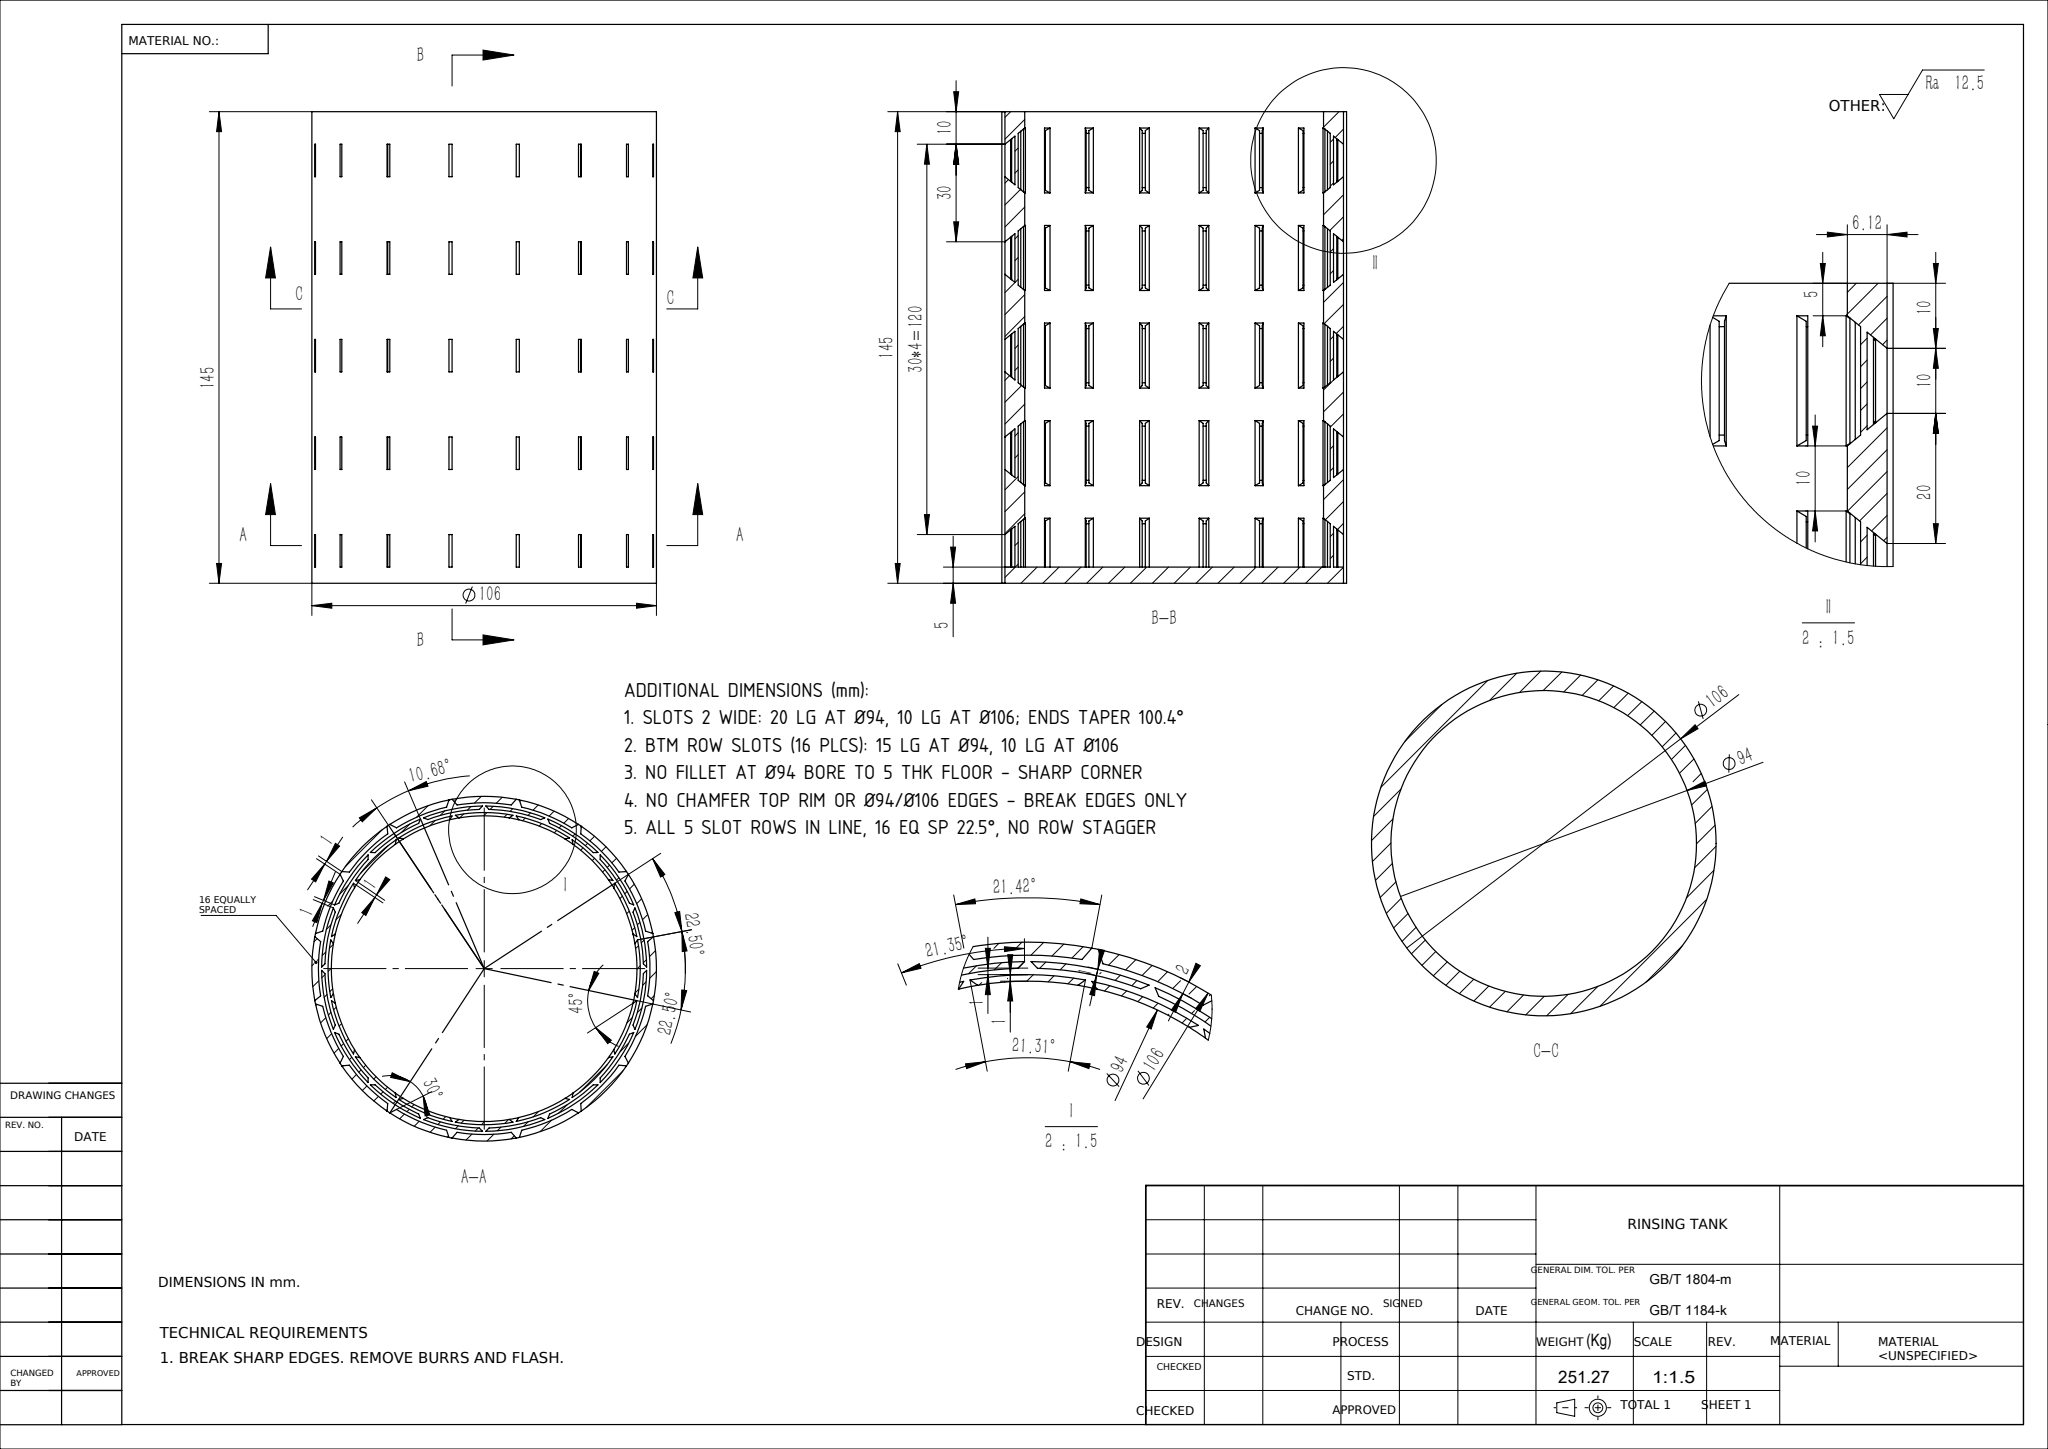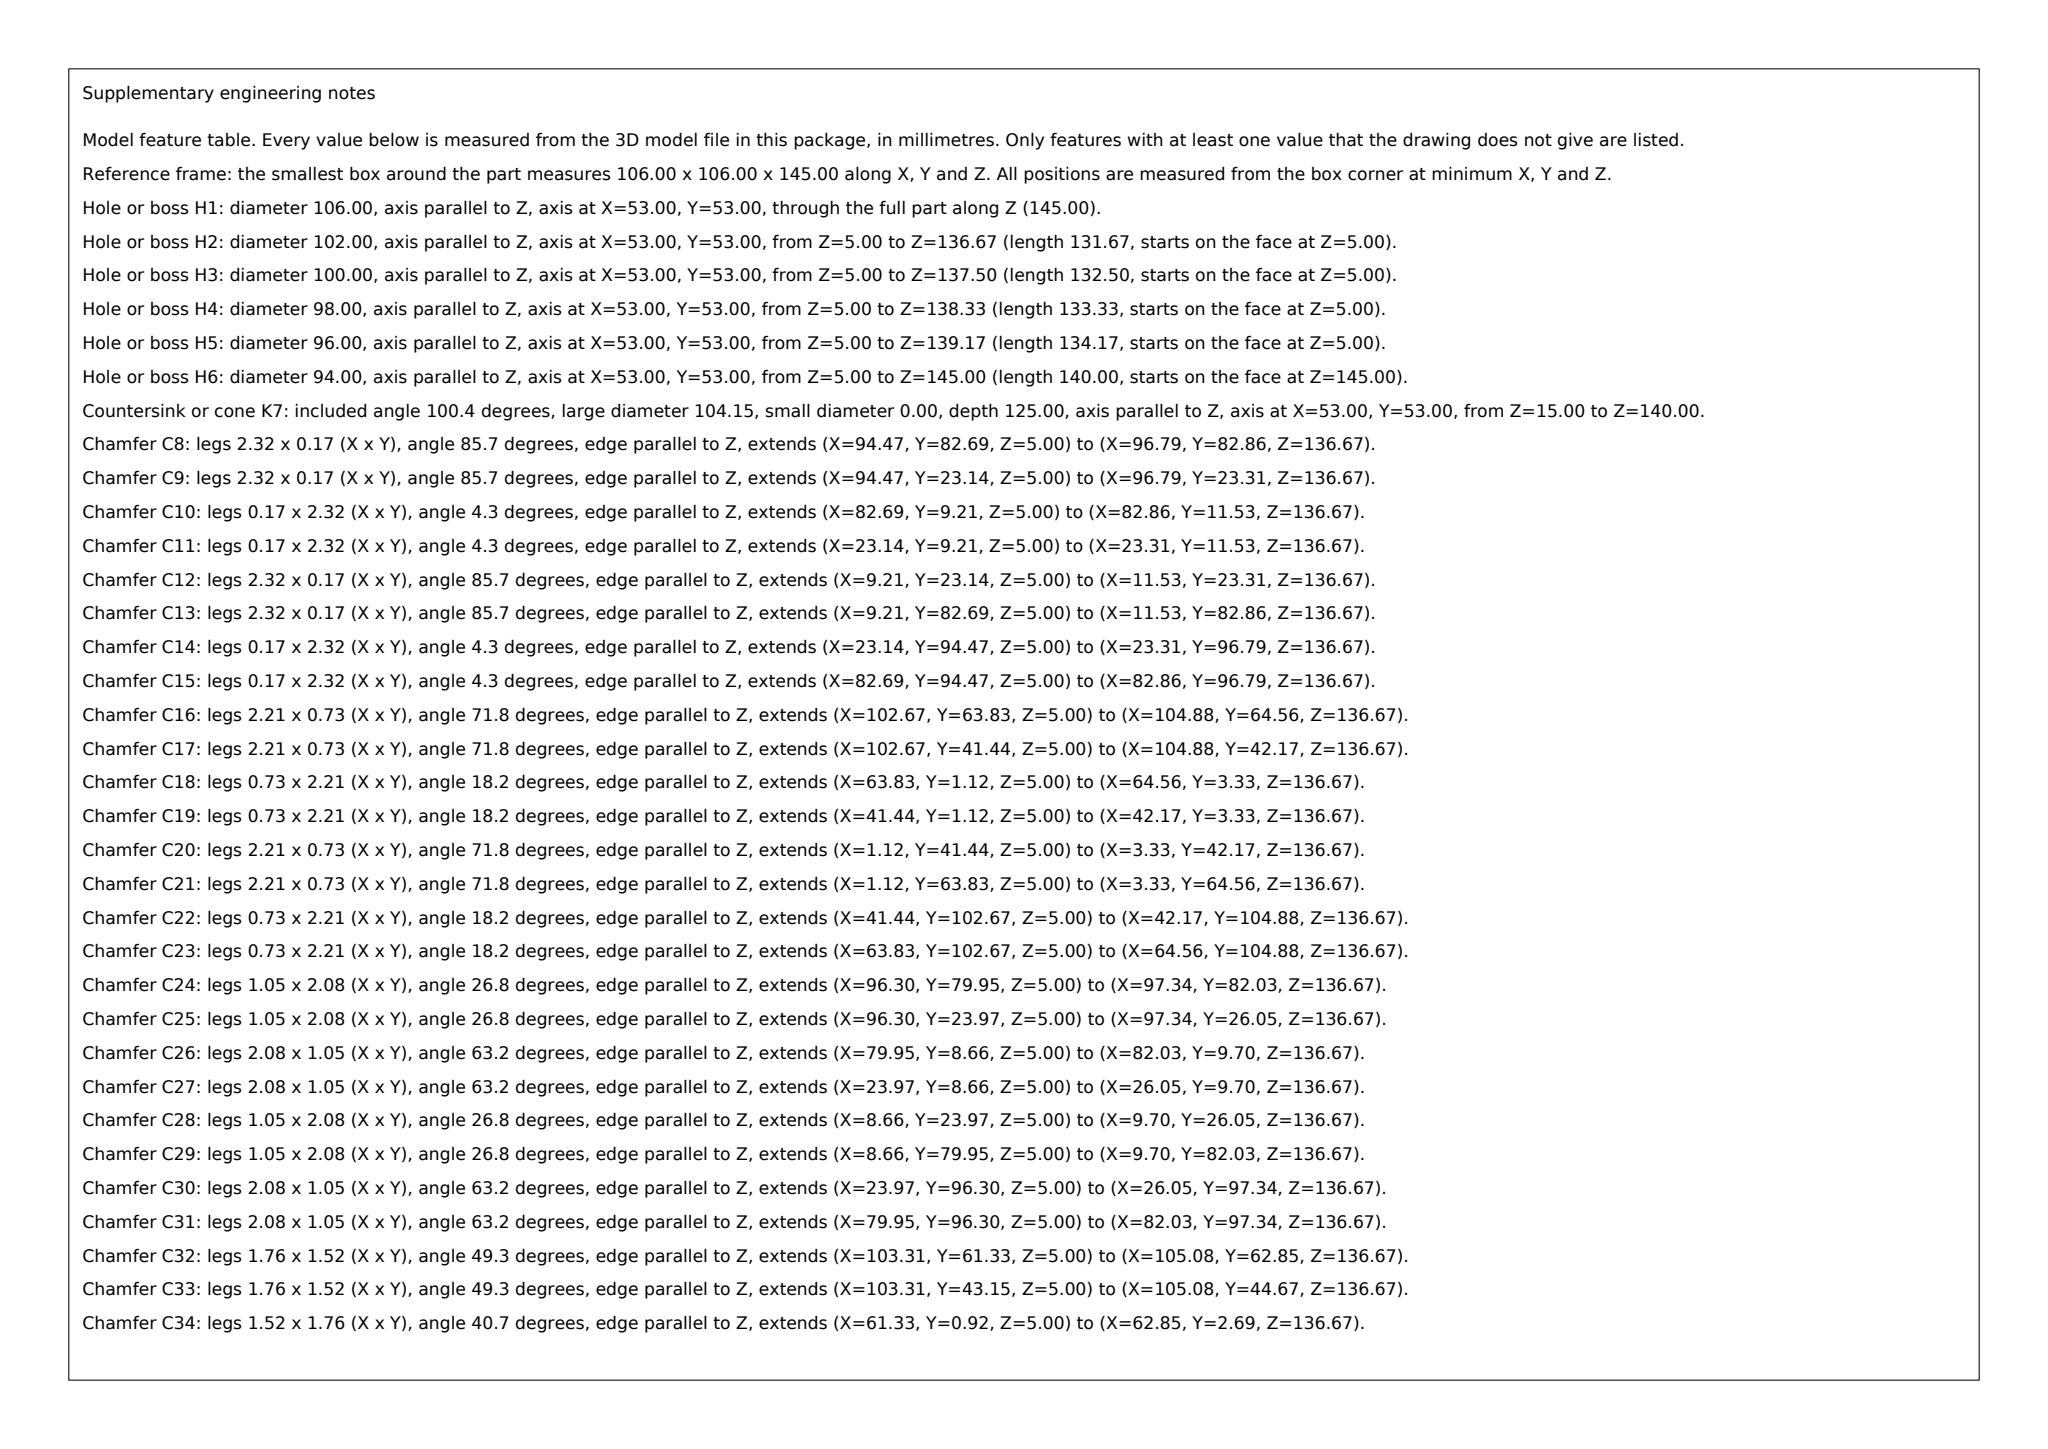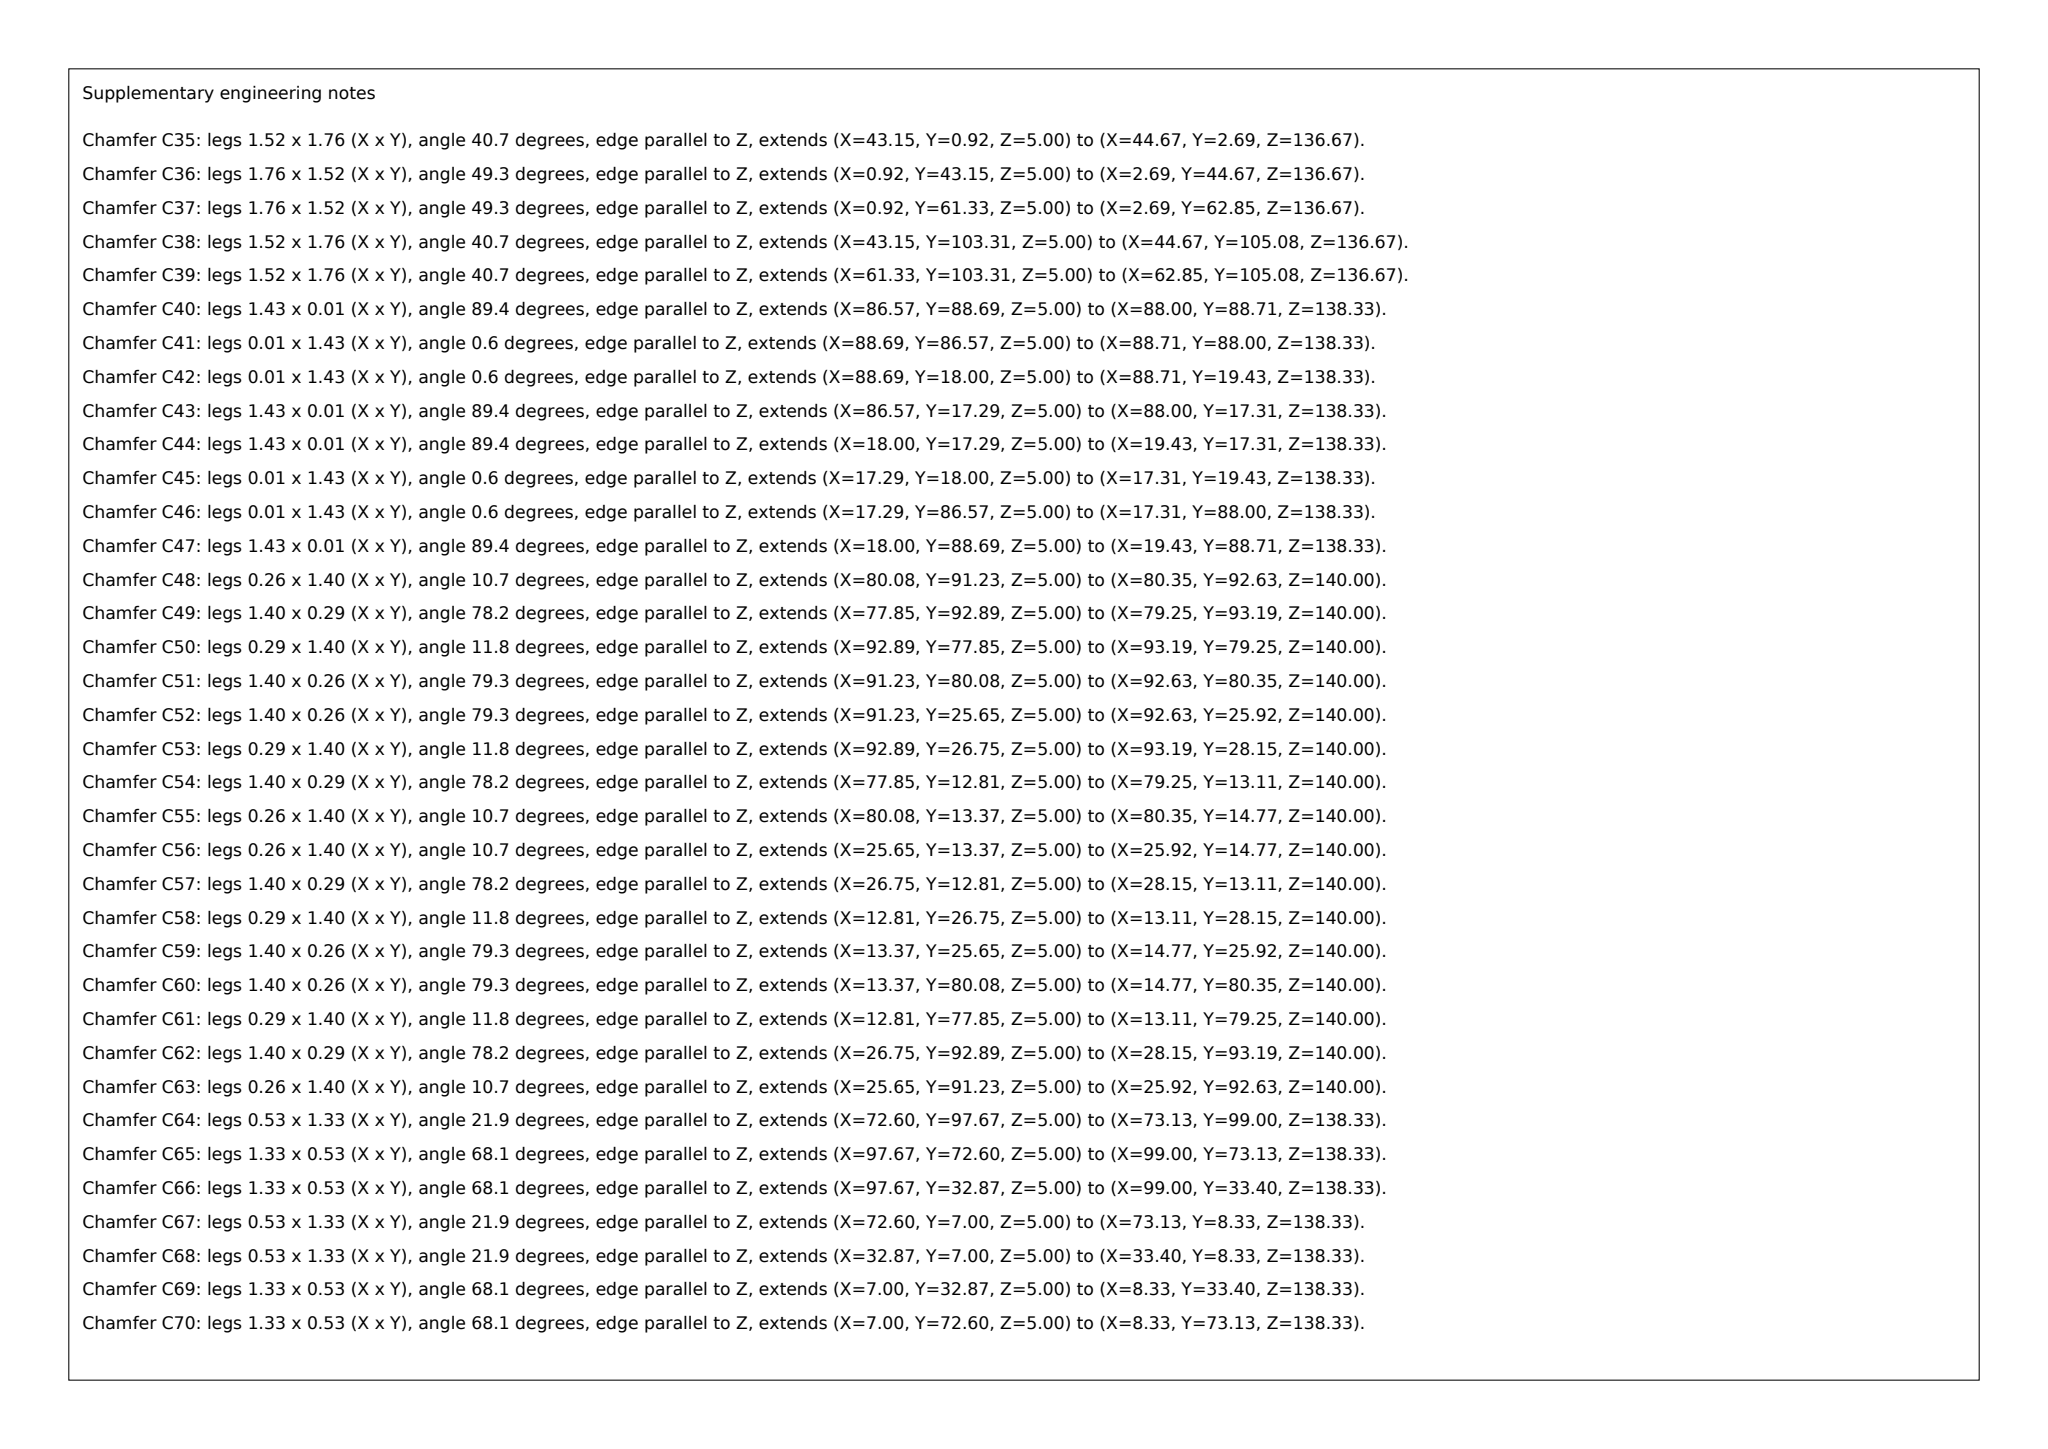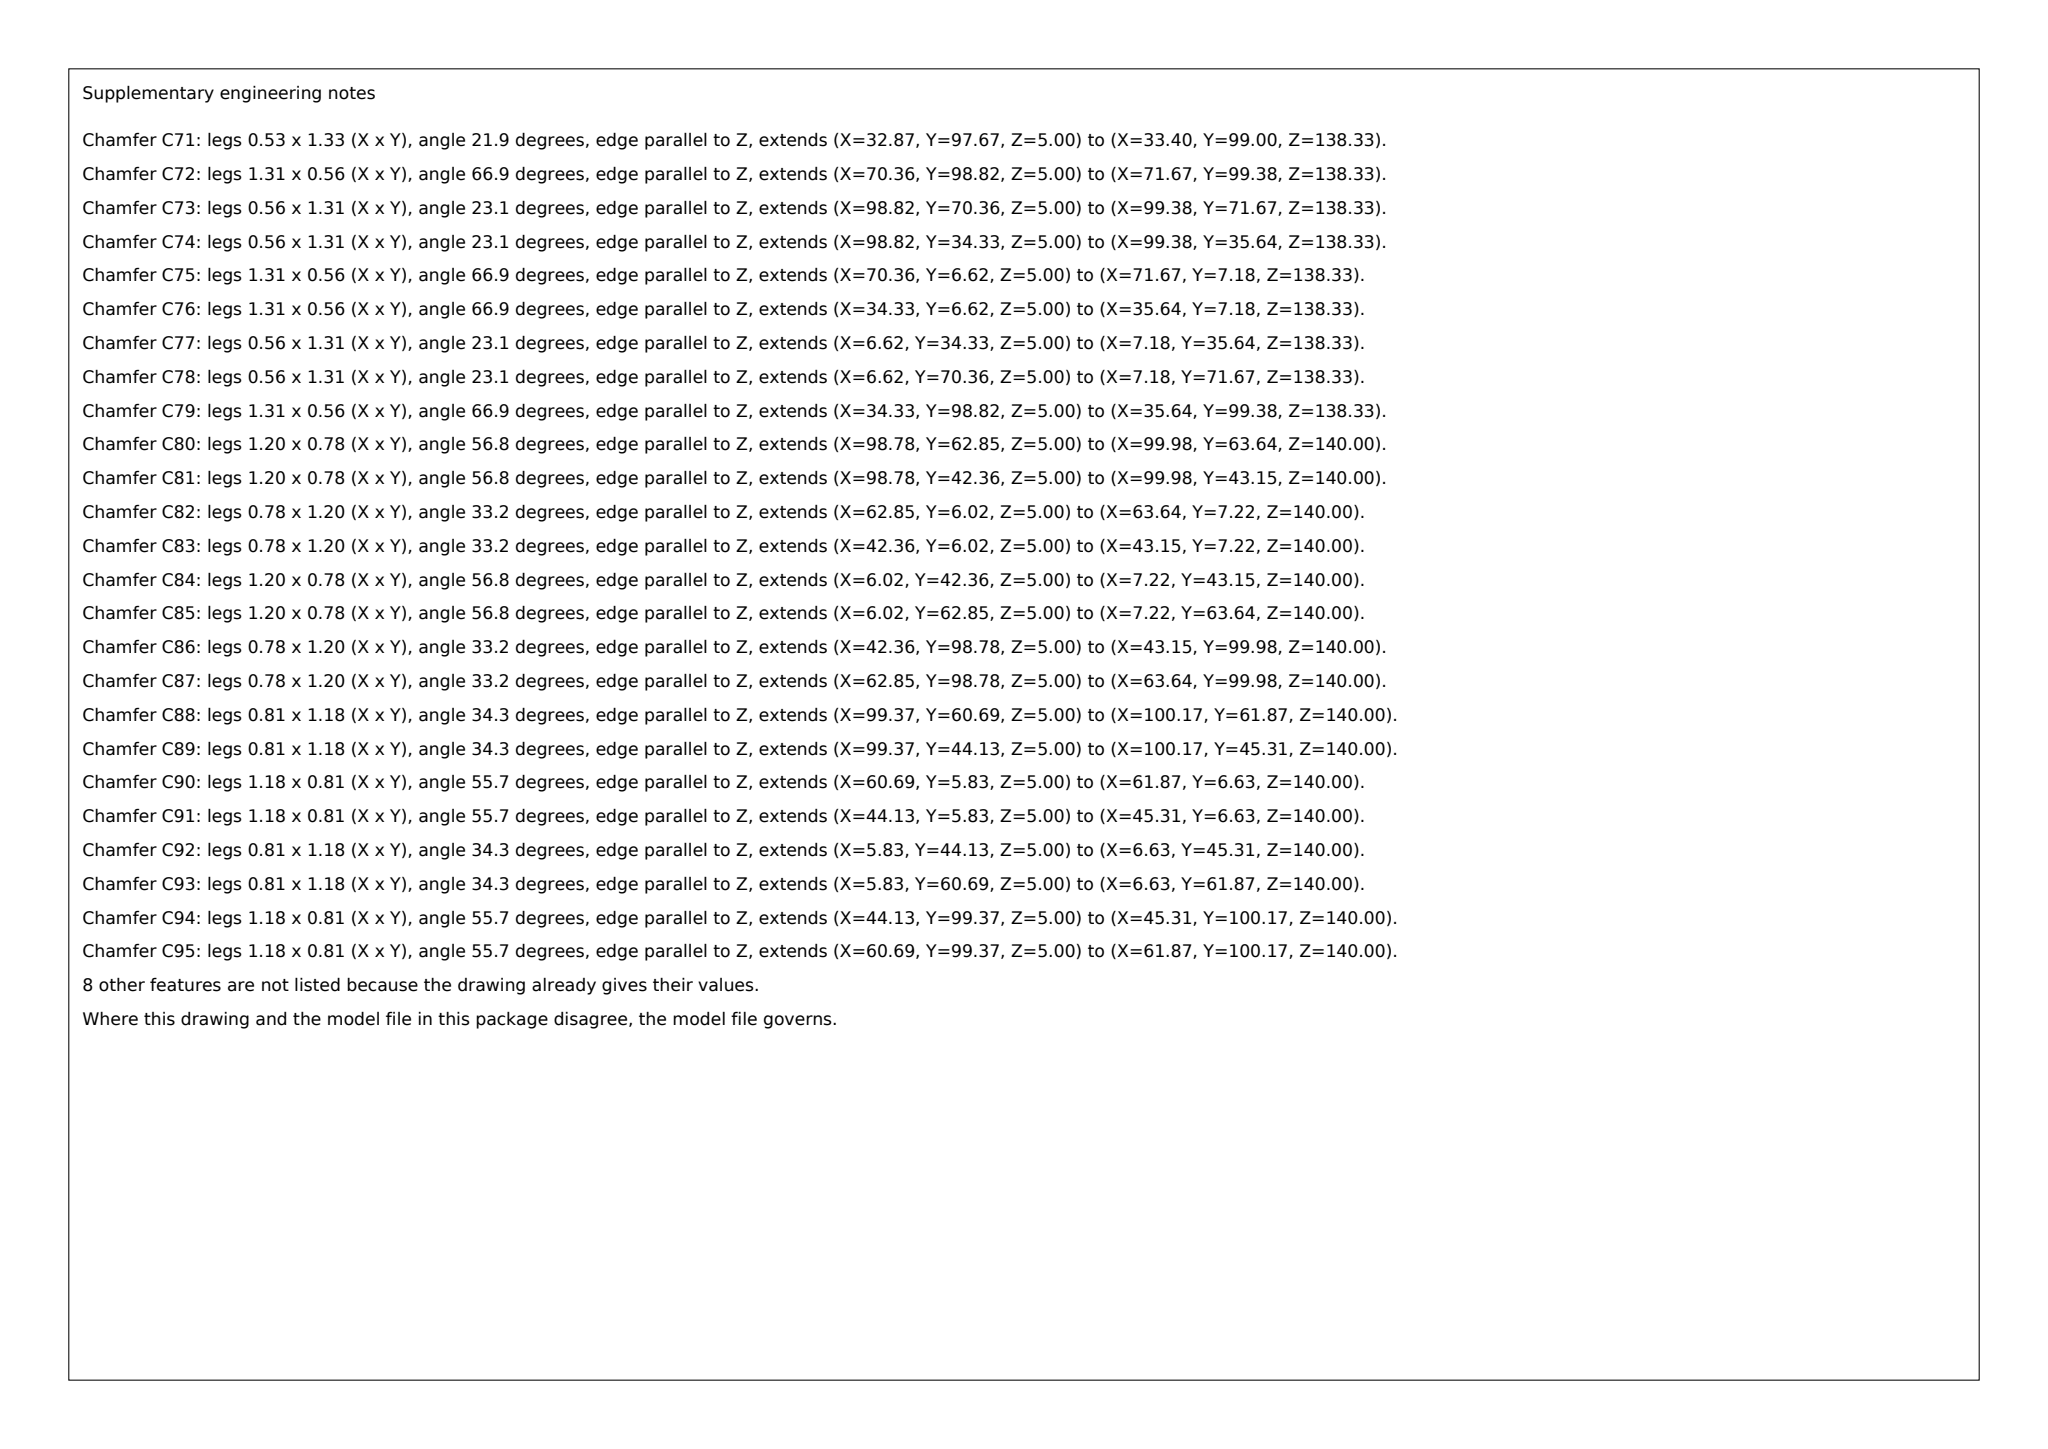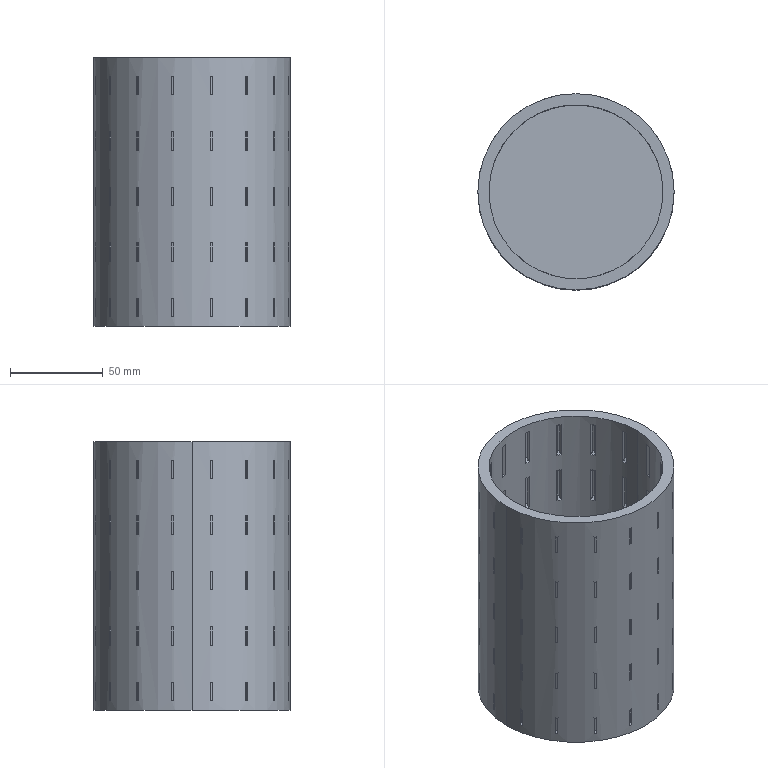Part | SolidWorks | mm | 1 solid | 825 faces | box 106 x 106 x 145 mm | volume 251267 mm3 | plane 483 | cylinder 324 | cone 18 | commonest cylinder face diameters 100 x80 98 x80 102 x80 96 x80 106 x2 94 x2